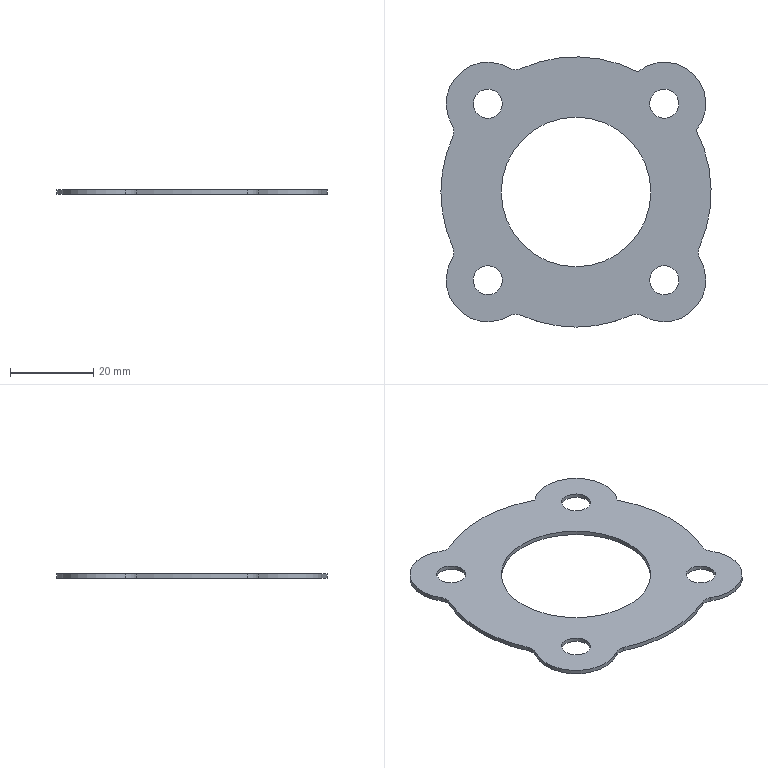Component | NX | GASKET | 1 solid | 21 faces | volume 2619 mm3 | cylinder 19 | plane 2 | commonest cylinder face diameters 6 x6 20 x4 65 x4 7 x4 36 x1